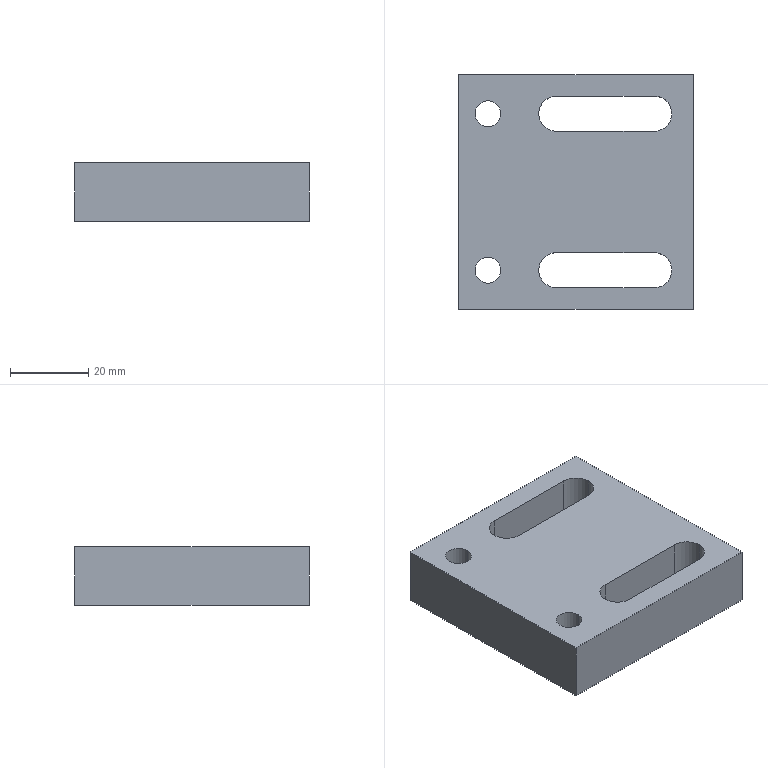Component | SolidWorks | CylinderSupportFrame01-1 | 1 solid | 26 faces | box 60 x 60 x 15 mm | volume 43488 mm3 | cylinder 14 | plane 12 | commonest cylinder face diameters 9 x6 11 x4 6.6 x4
build123d program:
from build123d import *

# Parameters (mm, degrees)
BOSS_EXTRUDE1_DEPTH                               = 60
SKETCH2_W                                         = 105
SKETCH2_H                                         = 15
BOSS_EXTRUDE2_DEPTH                               = 30
SKETCH5_W                                         = 111.678
SKETCH5_H                                         = 197
CUT_EXTRUDE1_DEPTH                                = 275.853
HOLE_SIZE_ACCORDING_TO_TYPE_OF_HEX_SO_D           = 6.6
HOLE_SIZE_ACCORDING_TO_TYPE_OF_HEX_SO_CBORE_D     = 11
HOLE_SIZE_ACCORDING_TO_TYPE_OF_HEX_SO_CBORE_DEPTH = 6.8
CUT_EXTRUDE2_DEPTH                                = 122.861


with BuildPart() as part:
    # Sketch1 → Boss-Extrude1 (new body)
    with BuildSketch(Plane(origin=(0, 0, 0), x_dir=(1, 0, 0), z_dir=(0, 1, 0))):
        Polygon((45, 0), (105, 0), (105, -15), (60, -15), (60, -197), (150, -197), (150, -212), (45, -212), align=None)
    extrude(amount=BOSS_EXTRUDE1_DEPTH)

    # Sketch2 → Boss-Extrude2 (add)
    with BuildSketch(Plane.XZ):
        with Locations((97.5, 204.5)):
            Rectangle(SKETCH2_W, SKETCH2_H)
    extrude(amount=BOSS_EXTRUDE2_DEPTH)

    # Sketch5 → Cut-Extrude1 (cut, through all)
    with BuildSketch(Plane(origin=(0, 60, 0), x_dir=(1, 0, 0), z_dir=(0, 1, 0))):
        with Locations((94.161, -113.5)):
            Rectangle(SKETCH5_W, SKETCH5_H)
    extrude(amount=-CUT_EXTRUDE1_DEPTH, mode=Mode.SUBTRACT)

    # Hole Size _ according to_ type of Hex So (through all)
    with Locations(Plane(origin=(52.5, 50, 0), x_dir=(-1, 0, 0), z_dir=(0, 0, -1))):
        with Locations((0, 0), (0, -40)):
            CounterBoreHole(HOLE_SIZE_ACCORDING_TO_TYPE_OF_HEX_SO_D / 2, HOLE_SIZE_ACCORDING_TO_TYPE_OF_HEX_SO_CBORE_D / 2, HOLE_SIZE_ACCORDING_TO_TYPE_OF_HEX_SO_CBORE_DEPTH)

    # Sketch7 → Cut-Extrude2 (cut, through all)
    with BuildSketch(Plane.XY.offset(15)):
        with BuildLine():
            Line((95, 5.5), (70, 5.5))
            ThreePointArc((70, 5.5), (65.5, 10), (70, 14.5))
            Line((70, 14.5), (95, 14.5))
            ThreePointArc((95, 14.5), (99.5, 10), (95, 5.5))
        make_face()
    cut_extrude2 = extrude(amount=-CUT_EXTRUDE2_DEPTH, mode=Mode.SUBTRACT)

    # Mirror1: Cut-Extrude2 across plane
    add(cut_extrude2.mirror(Plane.ZX.offset(30)), mode=Mode.SUBTRACT)


solid = part.part

# Placed as in the assembly
solid = solid.moved(Location((-44.66, -15.234, 43.104), (0, 0, 0)))
STEP:
#1=CARTESIAN_POINT('',(1.982,1.546,1.697));
#2=VERTEX_POINT('',#1);
#3=CARTESIAN_POINT('',(2.159,1.369,1.697));
#4=VERTEX_POINT('',#3);
#5=CARTESIAN_POINT('',(1.982,1.369,1.697));
#6=DIRECTION('',(0.,0.,-1.));
#7=DIRECTION('',(1.,0.,0.));
#8=AXIS2_PLACEMENT_3D('',#5,#6,#7);
#9=CIRCLE('',#8,0.1772);
#10=EDGE_CURVE('',#2,#4,#9,.T.);
#11=ORIENTED_EDGE('',*,*,#10,.T.);
#12=CARTESIAN_POINT('',(2.159,1.369,2.288));
#13=VERTEX_POINT('',#12);
#14=CARTESIAN_POINT('',(2.159,1.369,1.697));
#15=DIRECTION('',(0.,0.,1.));
#16=VECTOR('',#15,39.37);
#17=LINE('',#14,#16);
#18=EDGE_CURVE('',#4,#13,#17,.T.);
#19=ORIENTED_EDGE('',*,*,#18,.T.);
#20=CARTESIAN_POINT('',(1.982,1.546,2.288));
#21=VERTEX_POINT('',#20);
#22=CARTESIAN_POINT('',(1.982,1.369,2.288));
#23=DIRECTION('',(0.,0.,-1.));
#24=DIRECTION('',(1.,0.,0.));
#25=AXIS2_PLACEMENT_3D('',#22,#23,#24);
#26=CIRCLE('',#25,0.1772);
#27=EDGE_CURVE('',#21,#13,#26,.T.);
#28=ORIENTED_EDGE('',*,*,#27,.F.);
#29=CARTESIAN_POINT('',(1.982,1.546,1.697));
#30=DIRECTION('',(0.,0.,1.));
#31=VECTOR('',#30,39.37);
#32=LINE('',#29,#31);
#33=EDGE_CURVE('',#2,#21,#32,.T.);
#34=ORIENTED_EDGE('',*,*,#33,.F.);
#35=EDGE_LOOP('',(#11,#19,#28,#34));
#36=FACE_OUTER_BOUND('',#35,.T.);
#37=CARTESIAN_POINT('',(1.982,1.369,1.697));
#38=DIRECTION('',(0.,0.,1.));
#39=DIRECTION('',(1.,0.,0.));
#40=AXIS2_PLACEMENT_3D('',#37,#38,#39);
#41=CYLINDRICAL_SURFACE('',#40,0.1772);
#42=ADVANCED_FACE('',(#36),#41,.F.);
#43=CARTESIAN_POINT('',(2.159,-0.2061,1.697));
#44=VERTEX_POINT('',#43);
#45=CARTESIAN_POINT('',(1.982,-0.0289,1.697));
#46=VERTEX_POINT('',#45);
#47=CARTESIAN_POINT('',(1.982,-0.2061,1.697));
#48=DIRECTION('',(0.,0.,1.));
#49=DIRECTION('',(1.,0.,0.));
#50=AXIS2_PLACEMENT_3D('',#47,#48,#49);
#51=CIRCLE('',#50,0.1772);
#52=EDGE_CURVE('',#44,#46,#51,.T.);
#53=ORIENTED_EDGE('',*,*,#52,.F.);
#54=CARTESIAN_POINT('',(2.159,-0.2061,2.288));
#55=VERTEX_POINT('',#54);
#56=CARTESIAN_POINT('',(2.159,-0.2061,1.697));
#57=DIRECTION('',(0.,0.,1.));
#58=VECTOR('',#57,39.37);
#59=LINE('',#56,#58);
#60=EDGE_CURVE('',#44,#55,#59,.T.);
#61=ORIENTED_EDGE('',*,*,#60,.T.);
#62=CARTESIAN_POINT('',(1.982,-0.0289,2.288));
#63=VERTEX_POINT('',#62);
#64=CARTESIAN_POINT('',(1.982,-0.2061,2.288));
#65=DIRECTION('',(0.,0.,1.));
#66=DIRECTION('',(1.,0.,0.));
#67=AXIS2_PLACEMENT_3D('',#64,#65,#66);
#68=CIRCLE('',#67,0.1772);
#69=EDGE_CURVE('',#55,#63,#68,.T.);
#70=ORIENTED_EDGE('',*,*,#69,.T.);
#71=CARTESIAN_POINT('',(1.982,-0.0289,1.697));
#72=DIRECTION('',(0.,0.,1.));
#73=VECTOR('',#72,39.37);
#74=LINE('',#71,#73);
#75=EDGE_CURVE('',#46,#63,#74,.T.);
#76=ORIENTED_EDGE('',*,*,#75,.F.);
#77=EDGE_LOOP('',(#53,#61,#70,#76));
#78=FACE_OUTER_BOUND('',#77,.T.);
#79=CARTESIAN_POINT('',(1.982,-0.2061,1.697));
#80=DIRECTION('',(0.,0.,1.));
#81=DIRECTION('',(1.,0.,0.));
#82=AXIS2_PLACEMENT_3D('',#79,#80,#81);
#83=CYLINDRICAL_SURFACE('',#82,0.1772);
#84=ADVANCED_FACE('',(#78),#83,.F.);
#85=CARTESIAN_POINT('',(0.5252,1.369,1.965));
#86=VERTEX_POINT('',#85);
#87=CARTESIAN_POINT('',(0.09214,1.369,1.965));
#88=VERTEX_POINT('',#87);
#89=CARTESIAN_POINT('',(0.3087,1.369,1.965));
#90=DIRECTION('',(0.,0.,-1.));
#91=DIRECTION('',(-1.,0.,0.));
#92=AXIS2_PLACEMENT_3D('',#89,#90,#91);
#93=CIRCLE('',#92,0.2165);
#94=EDGE_CURVE('',#86,#88,#93,.T.);
#95=ORIENTED_EDGE('',*,*,#94,.F.);
#96=CARTESIAN_POINT('',(0.5252,1.369,1.697));
#97=VERTEX_POINT('',#96);
#98=CARTESIAN_POINT('',(0.5252,1.369,1.697));
#99=DIRECTION('',(0.,0.,-1.));
#100=VECTOR('',#99,39.37);
#101=LINE('',#98,#100);
#102=EDGE_CURVE('',#86,#97,#101,.T.);
#103=ORIENTED_EDGE('',*,*,#102,.T.);
#104=CARTESIAN_POINT('',(0.09214,1.369,1.697));
#105=VERTEX_POINT('',#104);
#106=CARTESIAN_POINT('',(0.3087,1.369,1.697));
#107=DIRECTION('',(0.,0.,-1.));
#108=DIRECTION('',(-1.,0.,0.));
#109=AXIS2_PLACEMENT_3D('',#106,#107,#108);
#110=CIRCLE('',#109,0.2165);
#111=EDGE_CURVE('',#97,#105,#110,.T.);
#112=ORIENTED_EDGE('',*,*,#111,.T.);
#113=CARTESIAN_POINT('',(0.09214,1.369,1.697));
#114=DIRECTION('',(0.,0.,-1.));
#115=VECTOR('',#114,39.37);
#116=LINE('',#113,#115);
#117=EDGE_CURVE('',#88,#105,#116,.T.);
#118=ORIENTED_EDGE('',*,*,#117,.F.);
#119=EDGE_LOOP('',(#95,#103,#112,#118));
#120=FACE_OUTER_BOUND('',#119,.T.);
#121=CARTESIAN_POINT('',(0.3087,1.369,1.697));
#122=DIRECTION('',(0.,0.,-1.));
#123=DIRECTION('',(-1.,0.,0.));
#124=AXIS2_PLACEMENT_3D('',#121,#122,#123);
#125=CYLINDRICAL_SURFACE('',#124,0.2165);
#126=ADVANCED_FACE('',(#120),#125,.F.);
#127=CARTESIAN_POINT('',(0.4386,1.369,2.288));
#128=VERTEX_POINT('',#127);
#129=CARTESIAN_POINT('',(0.1788,1.369,2.288));
#130=VERTEX_POINT('',#129);
#131=CARTESIAN_POINT('',(0.3087,1.369,2.288));
#132=DIRECTION('',(0.,0.,-1.));
#133=DIRECTION('',(-1.,0.,0.));
#134=AXIS2_PLACEMENT_3D('',#131,#132,#133);
#135=CIRCLE('',#134,0.1299);
#136=EDGE_CURVE('',#128,#130,#135,.T.);
#137=ORIENTED_EDGE('',*,*,#136,.F.);
#138=CARTESIAN_POINT('',(0.4386,1.369,1.965));
#139=VERTEX_POINT('',#138);
#140=CARTESIAN_POINT('',(0.4386,1.369,1.697));
#141=DIRECTION('',(0.,0.,-1.));
#142=VECTOR('',#141,39.37);
#143=LINE('',#140,#142);
#144=EDGE_CURVE('',#128,#139,#143,.T.);
#145=ORIENTED_EDGE('',*,*,#144,.T.);
#146=CARTESIAN_POINT('',(0.1788,1.369,1.965));
#147=VERTEX_POINT('',#146);
#148=CARTESIAN_POINT('',(0.3087,1.369,1.965));
#149=DIRECTION('',(0.,0.,-1.));
#150=DIRECTION('',(-1.,0.,0.));
#151=AXIS2_PLACEMENT_3D('',#148,#149,#150);
#152=CIRCLE('',#151,0.1299);
#153=EDGE_CURVE('',#139,#147,#152,.T.);
#154=ORIENTED_EDGE('',*,*,#153,.T.);
#155=CARTESIAN_POINT('',(0.1788,1.369,1.697));
#156=DIRECTION('',(0.,0.,-1.));
#157=VECTOR('',#156,39.37);
#158=LINE('',#155,#157);
#159=EDGE_CURVE('',#130,#147,#158,.T.);
#160=ORIENTED_EDGE('',*,*,#159,.F.);
#161=EDGE_LOOP('',(#137,#145,#154,#160));
#162=FACE_OUTER_BOUND('',#161,.T.);
#163=CARTESIAN_POINT('',(0.3087,1.369,1.697));
#164=DIRECTION('',(0.,0.,-1.));
#165=DIRECTION('',(-1.,0.,0.));
#166=AXIS2_PLACEMENT_3D('',#163,#164,#165);
#167=CYLINDRICAL_SURFACE('',#166,0.1299);
#168=ADVANCED_FACE('',(#162),#167,.F.);
#169=CARTESIAN_POINT('',(0.5252,-0.2061,1.965));
#170=VERTEX_POINT('',#169);
#171=CARTESIAN_POINT('',(0.09214,-0.2061,1.965));
#172=VERTEX_POINT('',#171);
#173=CARTESIAN_POINT('',(0.3087,-0.2061,1.965));
#174=DIRECTION('',(0.,0.,-1.));
#175=DIRECTION('',(-1.,0.,0.));
#176=AXIS2_PLACEMENT_3D('',#173,#174,#175);
#177=CIRCLE('',#176,0.2165);
#178=EDGE_CURVE('',#170,#172,#177,.T.);
#179=ORIENTED_EDGE('',*,*,#178,.F.);
#180=CARTESIAN_POINT('',(0.5252,-0.2061,1.697));
#181=VERTEX_POINT('',#180);
#182=CARTESIAN_POINT('',(0.5252,-0.2061,1.697));
#183=DIRECTION('',(0.,0.,-1.));
#184=VECTOR('',#183,39.37);
#185=LINE('',#182,#184);
#186=EDGE_CURVE('',#170,#181,#185,.T.);
#187=ORIENTED_EDGE('',*,*,#186,.T.);
#188=CARTESIAN_POINT('',(0.09214,-0.2061,1.697));
#189=VERTEX_POINT('',#188);
#190=CARTESIAN_POINT('',(0.3087,-0.2061,1.697));
#191=DIRECTION('',(0.,0.,-1.));
#192=DIRECTION('',(-1.,0.,0.));
#193=AXIS2_PLACEMENT_3D('',#190,#191,#192);
#194=CIRCLE('',#193,0.2165);
#195=EDGE_CURVE('',#181,#189,#194,.T.);
#196=ORIENTED_EDGE('',*,*,#195,.T.);
#197=CARTESIAN_POINT('',(0.09214,-0.2061,1.697));
#198=DIRECTION('',(0.,0.,-1.));
#199=VECTOR('',#198,39.37);
#200=LINE('',#197,#199);
#201=EDGE_CURVE('',#172,#189,#200,.T.);
#202=ORIENTED_EDGE('',*,*,#201,.F.);
#203=EDGE_LOOP('',(#179,#187,#196,#202));
#204=FACE_OUTER_BOUND('',#203,.T.);
#205=CARTESIAN_POINT('',(0.3087,-0.2061,1.697));
#206=DIRECTION('',(0.,0.,-1.));
#207=DIRECTION('',(-1.,0.,0.));
#208=AXIS2_PLACEMENT_3D('',#205,#206,#207);
#209=CYLINDRICAL_SURFACE('',#208,0.2165);
#210=ADVANCED_FACE('',(#204),#209,.F.);
#211=CARTESIAN_POINT('',(0.4386,-0.2061,2.288));
#212=VERTEX_POINT('',#211);
#213=CARTESIAN_POINT('',(0.1788,-0.2061,2.288));
#214=VERTEX_POINT('',#213);
#215=CARTESIAN_POINT('',(0.3087,-0.2061,2.288));
#216=DIRECTION('',(0.,0.,-1.));
#217=DIRECTION('',(-1.,0.,0.));
#218=AXIS2_PLACEMENT_3D('',#215,#216,#217);
#219=CIRCLE('',#218,0.1299);
#220=EDGE_CURVE('',#212,#214,#219,.T.);
#221=ORIENTED_EDGE('',*,*,#220,.F.);
#222=CARTESIAN_POINT('',(0.4386,-0.2061,1.965));
#223=VERTEX_POINT('',#222);
#224=CARTESIAN_POINT('',(0.4386,-0.2061,1.697));
#225=DIRECTION('',(0.,0.,-1.));
#226=VECTOR('',#225,39.37);
#227=LINE('',#224,#226);
#228=EDGE_CURVE('',#212,#223,#227,.T.);
#229=ORIENTED_EDGE('',*,*,#228,.T.);
#230=CARTESIAN_POINT('',(0.1788,-0.2061,1.965));
#231=VERTEX_POINT('',#230);
#232=CARTESIAN_POINT('',(0.3087,-0.2061,1.965));
#233=DIRECTION('',(0.,0.,-1.));
#234=DIRECTION('',(-1.,0.,0.));
#235=AXIS2_PLACEMENT_3D('',#232,#233,#234);
#236=CIRCLE('',#235,0.1299);
#237=EDGE_CURVE('',#223,#231,#236,.T.);
#238=ORIENTED_EDGE('',*,*,#237,.T.);
#239=CARTESIAN_POINT('',(0.1788,-0.2061,1.697));
#240=DIRECTION('',(0.,0.,-1.));
#241=VECTOR('',#240,39.37);
#242=LINE('',#239,#241);
#243=EDGE_CURVE('',#214,#231,#242,.T.);
#244=ORIENTED_EDGE('',*,*,#243,.F.);
#245=EDGE_LOOP('',(#221,#229,#238,#244));
#246=FACE_OUTER_BOUND('',#245,.T.);
#247=CARTESIAN_POINT('',(0.3087,-0.2061,1.697));
#248=DIRECTION('',(0.,0.,-1.));
#249=DIRECTION('',(-1.,0.,0.));
#250=AXIS2_PLACEMENT_3D('',#247,#248,#249);
#251=CYLINDRICAL_SURFACE('',#250,0.1299);
#252=ADVANCED_FACE('',(#246),#251,.F.);
#253=CARTESIAN_POINT('',(0.0134,-0.5998,2.288));
#254=VERTEX_POINT('',#253);
#255=CARTESIAN_POINT('',(2.376,-0.5998,2.288));
#256=VERTEX_POINT('',#255);
#257=CARTESIAN_POINT('',(0.604,-0.5998,2.288));
#258=DIRECTION('',(1.,0.,0.));
#259=VECTOR('',#258,39.37);
#260=LINE('',#257,#259);
#261=EDGE_CURVE('',#254,#256,#260,.T.);
#262=ORIENTED_EDGE('',*,*,#261,.T.);
#263=CARTESIAN_POINT('',(2.376,1.762,2.288));
#264=VERTEX_POINT('',#263);
#265=CARTESIAN_POINT('',(2.376,1.762,2.288));
#266=DIRECTION('',(0.,-1.,0.));
#267=VECTOR('',#266,39.37);
#268=LINE('',#265,#267);
#269=EDGE_CURVE('',#264,#256,#268,.T.);
#270=ORIENTED_EDGE('',*,*,#269,.F.);
#271=CARTESIAN_POINT('',(0.0134,1.762,2.288));
#272=VERTEX_POINT('',#271);
#273=CARTESIAN_POINT('',(0.604,1.762,2.288));
#274=DIRECTION('',(1.,0.,0.));
#275=VECTOR('',#274,39.37);
#276=LINE('',#273,#275);
#277=EDGE_CURVE('',#272,#264,#276,.T.);
#278=ORIENTED_EDGE('',*,*,#277,.F.);
#279=CARTESIAN_POINT('',(0.0134,1.762,2.288));
#280=DIRECTION('',(0.,1.,0.));
#281=VECTOR('',#280,39.37);
#282=LINE('',#279,#281);
#283=EDGE_CURVE('',#254,#272,#282,.T.);
#284=ORIENTED_EDGE('',*,*,#283,.F.);
#285=EDGE_LOOP('',(#262,#270,#278,#284));
#286=FACE_OUTER_BOUND('',#285,.T.);
#287=CARTESIAN_POINT('',(0.3087,-0.2061,2.288));
#288=DIRECTION('',(0.,0.,-1.));
#289=DIRECTION('',(-1.,0.,0.));
#290=AXIS2_PLACEMENT_3D('',#287,#288,#289);
#291=CIRCLE('',#290,0.1299);
#292=EDGE_CURVE('',#214,#212,#291,.T.);
#293=ORIENTED_EDGE('',*,*,#292,.T.);
#294=ORIENTED_EDGE('',*,*,#220,.T.);
#295=EDGE_LOOP('',(#293,#294));
#296=FACE_BOUND('',#295,.T.);
#297=CARTESIAN_POINT('',(0.3087,1.369,2.288));
#298=DIRECTION('',(0.,0.,-1.));
#299=DIRECTION('',(-1.,0.,0.));
#300=AXIS2_PLACEMENT_3D('',#297,#298,#299);
#301=CIRCLE('',#300,0.1299);
#302=EDGE_CURVE('',#130,#128,#301,.T.);
#303=ORIENTED_EDGE('',*,*,#302,.T.);
#304=ORIENTED_EDGE('',*,*,#136,.T.);
#305=EDGE_LOOP('',(#303,#304));
#306=FACE_BOUND('',#305,.T.);
#307=CARTESIAN_POINT('',(0.9977,-0.0289,2.288));
#308=VERTEX_POINT('',#307);
#309=CARTESIAN_POINT('',(1.982,-0.0289,2.288));
#310=DIRECTION('',(-1.,-0.,0.));
#311=VECTOR('',#310,39.37);
#312=LINE('',#309,#311);
#313=EDGE_CURVE('',#63,#308,#312,.T.);
#314=ORIENTED_EDGE('',*,*,#313,.F.);
#315=ORIENTED_EDGE('',*,*,#69,.F.);
#316=CARTESIAN_POINT('',(1.982,-0.3832,2.288));
#317=VERTEX_POINT('',#316);
#318=CARTESIAN_POINT('',(1.982,-0.2061,2.288));
#319=DIRECTION('',(0.,0.,1.));
#320=DIRECTION('',(1.,0.,0.));
#321=AXIS2_PLACEMENT_3D('',#318,#319,#320);
#322=CIRCLE('',#321,0.1772);
#323=EDGE_CURVE('',#317,#55,#322,.T.);
#324=ORIENTED_EDGE('',*,*,#323,.F.);
#325=CARTESIAN_POINT('',(0.9977,-0.3832,2.288));
#326=VERTEX_POINT('',#325);
#327=CARTESIAN_POINT('',(1.982,-0.3832,2.288));
#328=DIRECTION('',(1.,0.,0.));
#329=VECTOR('',#328,39.37);
#330=LINE('',#327,#329);
#331=EDGE_CURVE('',#326,#317,#330,.T.);
#332=ORIENTED_EDGE('',*,*,#331,.F.);
#333=CARTESIAN_POINT('',(0.9977,-0.2061,2.288));
#334=DIRECTION('',(0.,0.,1.));
#335=DIRECTION('',(1.,0.,0.));
#336=AXIS2_PLACEMENT_3D('',#333,#334,#335);
#337=CIRCLE('',#336,0.1772);
#338=EDGE_CURVE('',#308,#326,#337,.T.);
#339=ORIENTED_EDGE('',*,*,#338,.F.);
#340=EDGE_LOOP('',(#314,#315,#324,#332,#339));
#341=FACE_BOUND('',#340,.T.);
#342=ORIENTED_EDGE('',*,*,#27,.T.);
#343=CARTESIAN_POINT('',(1.982,1.192,2.288));
#344=VERTEX_POINT('',#343);
#345=CARTESIAN_POINT('',(1.982,1.369,2.288));
#346=DIRECTION('',(0.,0.,-1.));
#347=DIRECTION('',(1.,0.,0.));
#348=AXIS2_PLACEMENT_3D('',#345,#346,#347);
#349=CIRCLE('',#348,0.1772);
#350=EDGE_CURVE('',#13,#344,#349,.T.);
#351=ORIENTED_EDGE('',*,*,#350,.T.);
#352=CARTESIAN_POINT('',(0.9977,1.192,2.288));
#353=VERTEX_POINT('',#352);
#354=CARTESIAN_POINT('',(1.982,1.192,2.288));
#355=DIRECTION('',(-1.,0.,0.));
#356=VECTOR('',#355,39.37);
#357=LINE('',#354,#356);
#358=EDGE_CURVE('',#344,#353,#357,.T.);
#359=ORIENTED_EDGE('',*,*,#358,.T.);
#360=CARTESIAN_POINT('',(0.9977,1.546,2.288));
#361=VERTEX_POINT('',#360);
#362=CARTESIAN_POINT('',(0.9977,1.369,2.288));
#363=DIRECTION('',(0.,0.,-1.));
#364=DIRECTION('',(1.,0.,0.));
#365=AXIS2_PLACEMENT_3D('',#362,#363,#364);
#366=CIRCLE('',#365,0.1772);
#367=EDGE_CURVE('',#353,#361,#366,.T.);
#368=ORIENTED_EDGE('',*,*,#367,.T.);
#369=CARTESIAN_POINT('',(1.982,1.546,2.288));
#370=DIRECTION('',(1.,-0.,0.));
#371=VECTOR('',#370,39.37);
#372=LINE('',#369,#371);
#373=EDGE_CURVE('',#361,#21,#372,.T.);
#374=ORIENTED_EDGE('',*,*,#373,.T.);
#375=EDGE_LOOP('',(#342,#351,#359,#368,#374));
#376=FACE_BOUND('',#375,.T.);
#377=CARTESIAN_POINT('',(0.604,1.762,2.288));
#378=DIRECTION('',(0.,0.,-1.));
#379=DIRECTION('',(-1.,0.,0.));
#380=AXIS2_PLACEMENT_3D('',#377,#378,#379);
#381=PLANE('',#380);
#382=ADVANCED_FACE('',(#286,#296,#306,#341,#376),#381,.F.);
#383=CARTESIAN_POINT('',(2.376,-0.5998,1.697));
#384=VERTEX_POINT('',#383);
#385=CARTESIAN_POINT('',(0.0134,-0.5998,1.697));
#386=VERTEX_POINT('',#385);
#387=CARTESIAN_POINT('',(0.0134,-0.5998,1.697));
#388=DIRECTION('',(-1.,0.,0.));
#389=VECTOR('',#388,39.37);
#390=LINE('',#387,#389);
#391=EDGE_CURVE('',#384,#386,#390,.T.);
#392=ORIENTED_EDGE('',*,*,#391,.T.);
#393=CARTESIAN_POINT('',(0.0134,1.762,1.697));
#394=VERTEX_POINT('',#393);
#395=CARTESIAN_POINT('',(0.0134,1.762,1.697));
#396=DIRECTION('',(0.,-1.,0.));
#397=VECTOR('',#396,39.37);
#398=LINE('',#395,#397);
#399=EDGE_CURVE('',#394,#386,#398,.T.);
#400=ORIENTED_EDGE('',*,*,#399,.F.);
#401=CARTESIAN_POINT('',(2.376,1.762,1.697));
#402=VERTEX_POINT('',#401);
#403=CARTESIAN_POINT('',(0.0134,1.762,1.697));
#404=DIRECTION('',(-1.,0.,0.));
#405=VECTOR('',#404,39.37);
#406=LINE('',#403,#405);
#407=EDGE_CURVE('',#402,#394,#406,.T.);
#408=ORIENTED_EDGE('',*,*,#407,.F.);
#409=CARTESIAN_POINT('',(2.376,1.762,1.697));
#410=DIRECTION('',(0.,-1.,0.));
#411=VECTOR('',#410,39.37);
#412=LINE('',#409,#411);
#413=EDGE_CURVE('',#402,#384,#412,.T.);
#414=ORIENTED_EDGE('',*,*,#413,.T.);
#415=EDGE_LOOP('',(#392,#400,#408,#414));
#416=FACE_OUTER_BOUND('',#415,.T.);
#417=CARTESIAN_POINT('',(0.3087,-0.2061,1.697));
#418=DIRECTION('',(0.,0.,-1.));
#419=DIRECTION('',(-1.,0.,0.));
#420=AXIS2_PLACEMENT_3D('',#417,#418,#419);
#421=CIRCLE('',#420,0.2165);
#422=EDGE_CURVE('',#189,#181,#421,.T.);
#423=ORIENTED_EDGE('',*,*,#422,.F.);
#424=ORIENTED_EDGE('',*,*,#195,.F.);
#425=EDGE_LOOP('',(#423,#424));
#426=FACE_BOUND('',#425,.T.);
#427=CARTESIAN_POINT('',(0.3087,1.369,1.697));
#428=DIRECTION('',(0.,0.,-1.));
#429=DIRECTION('',(-1.,0.,0.));
#430=AXIS2_PLACEMENT_3D('',#427,#428,#429);
#431=CIRCLE('',#430,0.2165);
#432=EDGE_CURVE('',#105,#97,#431,.T.);
#433=ORIENTED_EDGE('',*,*,#432,.F.);
#434=ORIENTED_EDGE('',*,*,#111,.F.);
#435=EDGE_LOOP('',(#433,#434));
#436=FACE_BOUND('',#435,.T.);
#437=CARTESIAN_POINT('',(0.9977,-0.3832,1.697));
#438=VERTEX_POINT('',#437);
#439=CARTESIAN_POINT('',(1.982,-0.3832,1.697));
#440=VERTEX_POINT('',#439);
#441=CARTESIAN_POINT('',(1.982,-0.3832,1.697));
#442=DIRECTION('',(1.,0.,0.));
#443=VECTOR('',#442,39.37);
#444=LINE('',#441,#443);
#445=EDGE_CURVE('',#438,#440,#444,.T.);
#446=ORIENTED_EDGE('',*,*,#445,.T.);
#447=CARTESIAN_POINT('',(1.982,-0.2061,1.697));
#448=DIRECTION('',(0.,0.,1.));
#449=DIRECTION('',(1.,0.,0.));
#450=AXIS2_PLACEMENT_3D('',#447,#448,#449);
#451=CIRCLE('',#450,0.1772);
#452=EDGE_CURVE('',#440,#44,#451,.T.);
#453=ORIENTED_EDGE('',*,*,#452,.T.);
#454=ORIENTED_EDGE('',*,*,#52,.T.);
#455=CARTESIAN_POINT('',(0.9977,-0.0289,1.697));
#456=VERTEX_POINT('',#455);
#457=CARTESIAN_POINT('',(1.982,-0.0289,1.697));
#458=DIRECTION('',(-1.,-0.,0.));
#459=VECTOR('',#458,39.37);
#460=LINE('',#457,#459);
#461=EDGE_CURVE('',#46,#456,#460,.T.);
#462=ORIENTED_EDGE('',*,*,#461,.T.);
#463=CARTESIAN_POINT('',(0.9977,-0.2061,1.697));
#464=DIRECTION('',(0.,0.,1.));
#465=DIRECTION('',(1.,0.,0.));
#466=AXIS2_PLACEMENT_3D('',#463,#464,#465);
#467=CIRCLE('',#466,0.1772);
#468=EDGE_CURVE('',#456,#438,#467,.T.);
#469=ORIENTED_EDGE('',*,*,#468,.T.);
#470=EDGE_LOOP('',(#446,#453,#454,#462,#469));
#471=FACE_BOUND('',#470,.T.);
#472=ORIENTED_EDGE('',*,*,#10,.F.);
#473=CARTESIAN_POINT('',(0.9977,1.546,1.697));
#474=VERTEX_POINT('',#473);
#475=CARTESIAN_POINT('',(1.982,1.546,1.697));
#476=DIRECTION('',(1.,-0.,0.));
#477=VECTOR('',#476,39.37);
#478=LINE('',#475,#477);
#479=EDGE_CURVE('',#474,#2,#478,.T.);
#480=ORIENTED_EDGE('',*,*,#479,.F.);
#481=CARTESIAN_POINT('',(0.9977,1.192,1.697));
#482=VERTEX_POINT('',#481);
#483=CARTESIAN_POINT('',(0.9977,1.369,1.697));
#484=DIRECTION('',(0.,0.,-1.));
#485=DIRECTION('',(1.,0.,0.));
#486=AXIS2_PLACEMENT_3D('',#483,#484,#485);
#487=CIRCLE('',#486,0.1772);
#488=EDGE_CURVE('',#482,#474,#487,.T.);
#489=ORIENTED_EDGE('',*,*,#488,.F.);
#490=CARTESIAN_POINT('',(1.982,1.192,1.697));
#491=VERTEX_POINT('',#490);
#492=CARTESIAN_POINT('',(1.982,1.192,1.697));
#493=DIRECTION('',(-1.,0.,0.));
#494=VECTOR('',#493,39.37);
#495=LINE('',#492,#494);
#496=EDGE_CURVE('',#491,#482,#495,.T.);
#497=ORIENTED_EDGE('',*,*,#496,.F.);
#498=CARTESIAN_POINT('',(1.982,1.369,1.697));
#499=DIRECTION('',(0.,0.,-1.));
#500=DIRECTION('',(1.,0.,0.));
#501=AXIS2_PLACEMENT_3D('',#498,#499,#500);
#502=CIRCLE('',#501,0.1772);
#503=EDGE_CURVE('',#4,#491,#502,.T.);
#504=ORIENTED_EDGE('',*,*,#503,.F.);
#505=EDGE_LOOP('',(#472,#480,#489,#497,#504));
#506=FACE_BOUND('',#505,.T.);
#507=CARTESIAN_POINT('',(0.0134,1.762,1.697));
#508=DIRECTION('',(0.,0.,1.));
#509=DIRECTION('',(1.,0.,0.));
#510=AXIS2_PLACEMENT_3D('',#507,#508,#509);
#511=PLANE('',#510);
#512=ADVANCED_FACE('',(#416,#426,#436,#471,#506),#511,.F.);
#513=CARTESIAN_POINT('',(2.376,-0.5998,2.288));
#514=DIRECTION('',(0.,0.,-1.));
#515=VECTOR('',#514,39.37);
#516=LINE('',#513,#515);
#517=EDGE_CURVE('',#256,#384,#516,.T.);
#518=ORIENTED_EDGE('',*,*,#517,.T.);
#519=ORIENTED_EDGE('',*,*,#413,.F.);
#520=CARTESIAN_POINT('',(2.376,1.762,2.288));
#521=DIRECTION('',(0.,0.,-1.));
#522=VECTOR('',#521,39.37);
#523=LINE('',#520,#522);
#524=EDGE_CURVE('',#264,#402,#523,.T.);
#525=ORIENTED_EDGE('',*,*,#524,.F.);
#526=ORIENTED_EDGE('',*,*,#269,.T.);
#527=EDGE_LOOP('',(#518,#519,#525,#526));
#528=FACE_OUTER_BOUND('',#527,.T.);
#529=CARTESIAN_POINT('',(2.376,1.762,2.288));
#530=DIRECTION('',(-1.,0.,0.));
#531=DIRECTION('',(0.,0.,1.));
#532=AXIS2_PLACEMENT_3D('',#529,#530,#531);
#533=PLANE('',#532);
#534=ADVANCED_FACE('',(#528),#533,.F.);
#535=CARTESIAN_POINT('',(0.0134,-0.5998,1.697));
#536=DIRECTION('',(0.,0.,1.));
#537=VECTOR('',#536,39.37);
#538=LINE('',#535,#537);
#539=EDGE_CURVE('',#386,#254,#538,.T.);
#540=ORIENTED_EDGE('',*,*,#539,.T.);
#541=ORIENTED_EDGE('',*,*,#283,.T.);
#542=CARTESIAN_POINT('',(0.0134,1.762,1.697));
#543=DIRECTION('',(0.,0.,1.));
#544=VECTOR('',#543,39.37);
#545=LINE('',#542,#544);
#546=EDGE_CURVE('',#394,#272,#545,.T.);
#547=ORIENTED_EDGE('',*,*,#546,.F.);
#548=ORIENTED_EDGE('',*,*,#399,.T.);
#549=EDGE_LOOP('',(#540,#541,#547,#548));
#550=FACE_OUTER_BOUND('',#549,.T.);
#551=CARTESIAN_POINT('',(0.0134,1.762,1.697));
#552=DIRECTION('',(1.,0.,-0.));
#553=DIRECTION('',(-0.,0.,-1.));
#554=AXIS2_PLACEMENT_3D('',#551,#552,#553);
#555=PLANE('',#554);
#556=ADVANCED_FACE('',(#550),#555,.F.);
#557=ORIENTED_EDGE('',*,*,#546,.T.);
#558=ORIENTED_EDGE('',*,*,#277,.T.);
#559=ORIENTED_EDGE('',*,*,#524,.T.);
#560=ORIENTED_EDGE('',*,*,#407,.T.);
#561=EDGE_LOOP('',(#557,#558,#559,#560));
#562=FACE_OUTER_BOUND('',#561,.T.);
#563=CARTESIAN_POINT('',(-1.758,1.762,1.697));
#564=DIRECTION('',(0.,-1.,0.));
#565=DIRECTION('',(0.,0.,-1.));
#566=AXIS2_PLACEMENT_3D('',#563,#564,#565);
#567=PLANE('',#566);
#568=ADVANCED_FACE('',(#562),#567,.F.);
#569=ORIENTED_EDGE('',*,*,#261,.F.);
#570=ORIENTED_EDGE('',*,*,#539,.F.);
#571=ORIENTED_EDGE('',*,*,#391,.F.);
#572=ORIENTED_EDGE('',*,*,#517,.F.);
#573=EDGE_LOOP('',(#569,#570,#571,#572));
#574=FACE_OUTER_BOUND('',#573,.T.);
#575=CARTESIAN_POINT('',(-1.758,-0.5998,1.697));
#576=DIRECTION('',(0.,-1.,0.));
#577=DIRECTION('',(0.,0.,-1.));
#578=AXIS2_PLACEMENT_3D('',#575,#576,#577);
#579=PLANE('',#578);
#580=ADVANCED_FACE('',(#574),#579,.T.);
#581=ORIENTED_EDGE('',*,*,#228,.F.);
#582=ORIENTED_EDGE('',*,*,#292,.F.);
#583=ORIENTED_EDGE('',*,*,#243,.T.);
#584=CARTESIAN_POINT('',(0.3087,-0.2061,1.965));
#585=DIRECTION('',(0.,0.,-1.));
#586=DIRECTION('',(-1.,0.,0.));
#587=AXIS2_PLACEMENT_3D('',#584,#585,#586);
#588=CIRCLE('',#587,0.1299);
#589=EDGE_CURVE('',#231,#223,#588,.T.);
#590=ORIENTED_EDGE('',*,*,#589,.T.);
#591=EDGE_LOOP('',(#581,#582,#583,#590));
#592=FACE_OUTER_BOUND('',#591,.T.);
#593=CARTESIAN_POINT('',(0.3087,-0.2061,1.697));
#594=DIRECTION('',(0.,0.,-1.));
#595=DIRECTION('',(-1.,0.,0.));
#596=AXIS2_PLACEMENT_3D('',#593,#594,#595);
#597=CYLINDRICAL_SURFACE('',#596,0.1299);
#598=ADVANCED_FACE('',(#592),#597,.F.);
#599=ORIENTED_EDGE('',*,*,#589,.F.);
#600=ORIENTED_EDGE('',*,*,#237,.F.);
#601=EDGE_LOOP('',(#599,#600));
#602=FACE_BOUND('',#601,.T.);
#603=CARTESIAN_POINT('',(0.3087,-0.2061,1.965));
#604=DIRECTION('',(0.,0.,-1.));
#605=DIRECTION('',(-1.,0.,0.));
#606=AXIS2_PLACEMENT_3D('',#603,#604,#605);
#607=CIRCLE('',#606,0.2165);
#608=EDGE_CURVE('',#172,#170,#607,.T.);
#609=ORIENTED_EDGE('',*,*,#608,.T.);
#610=ORIENTED_EDGE('',*,*,#178,.T.);
#611=EDGE_LOOP('',(#609,#610));
#612=FACE_OUTER_BOUND('',#611,.T.);
#613=CARTESIAN_POINT('',(0.4386,-0.2061,1.965));
#614=DIRECTION('',(0.,0.,1.));
#615=DIRECTION('',(1.,0.,0.));
#616=AXIS2_PLACEMENT_3D('',#613,#614,#615);
#617=PLANE('',#616);
#618=ADVANCED_FACE('',(#602,#612),#617,.F.);
#619=ORIENTED_EDGE('',*,*,#186,.F.);
#620=ORIENTED_EDGE('',*,*,#608,.F.);
#621=ORIENTED_EDGE('',*,*,#201,.T.);
#622=ORIENTED_EDGE('',*,*,#422,.T.);
#623=EDGE_LOOP('',(#619,#620,#621,#622));
#624=FACE_OUTER_BOUND('',#623,.T.);
#625=CARTESIAN_POINT('',(0.3087,-0.2061,1.697));
#626=DIRECTION('',(0.,0.,-1.));
#627=DIRECTION('',(-1.,0.,0.));
#628=AXIS2_PLACEMENT_3D('',#625,#626,#627);
#629=CYLINDRICAL_SURFACE('',#628,0.2165);
#630=ADVANCED_FACE('',(#624),#629,.F.);
#631=ORIENTED_EDGE('',*,*,#144,.F.);
#632=ORIENTED_EDGE('',*,*,#302,.F.);
#633=ORIENTED_EDGE('',*,*,#159,.T.);
#634=CARTESIAN_POINT('',(0.3087,1.369,1.965));
#635=DIRECTION('',(0.,0.,-1.));
#636=DIRECTION('',(-1.,0.,0.));
#637=AXIS2_PLACEMENT_3D('',#634,#635,#636);
#638=CIRCLE('',#637,0.1299);
#639=EDGE_CURVE('',#147,#139,#638,.T.);
#640=ORIENTED_EDGE('',*,*,#639,.T.);
#641=EDGE_LOOP('',(#631,#632,#633,#640));
#642=FACE_OUTER_BOUND('',#641,.T.);
#643=CARTESIAN_POINT('',(0.3087,1.369,1.697));
#644=DIRECTION('',(0.,0.,-1.));
#645=DIRECTION('',(-1.,0.,0.));
#646=AXIS2_PLACEMENT_3D('',#643,#644,#645);
#647=CYLINDRICAL_SURFACE('',#646,0.1299);
#648=ADVANCED_FACE('',(#642),#647,.F.);
#649=ORIENTED_EDGE('',*,*,#639,.F.);
#650=ORIENTED_EDGE('',*,*,#153,.F.);
#651=EDGE_LOOP('',(#649,#650));
#652=FACE_BOUND('',#651,.T.);
#653=CARTESIAN_POINT('',(0.3087,1.369,1.965));
#654=DIRECTION('',(0.,0.,-1.));
#655=DIRECTION('',(-1.,0.,0.));
#656=AXIS2_PLACEMENT_3D('',#653,#654,#655);
#657=CIRCLE('',#656,0.2165);
#658=EDGE_CURVE('',#88,#86,#657,.T.);
#659=ORIENTED_EDGE('',*,*,#658,.T.);
#660=ORIENTED_EDGE('',*,*,#94,.T.);
#661=EDGE_LOOP('',(#659,#660));
#662=FACE_OUTER_BOUND('',#661,.T.);
#663=CARTESIAN_POINT('',(0.4386,1.369,1.965));
#664=DIRECTION('',(0.,0.,1.));
#665=DIRECTION('',(1.,0.,0.));
#666=AXIS2_PLACEMENT_3D('',#663,#664,#665);
#667=PLANE('',#666);
#668=ADVANCED_FACE('',(#652,#662),#667,.F.);
#669=ORIENTED_EDGE('',*,*,#102,.F.);
#670=ORIENTED_EDGE('',*,*,#658,.F.);
#671=ORIENTED_EDGE('',*,*,#117,.T.);
#672=ORIENTED_EDGE('',*,*,#432,.T.);
#673=EDGE_LOOP('',(#669,#670,#671,#672));
#674=FACE_OUTER_BOUND('',#673,.T.);
#675=CARTESIAN_POINT('',(0.3087,1.369,1.697));
#676=DIRECTION('',(0.,0.,-1.));
#677=DIRECTION('',(-1.,0.,0.));
#678=AXIS2_PLACEMENT_3D('',#675,#676,#677);
#679=CYLINDRICAL_SURFACE('',#678,0.2165);
#680=ADVANCED_FACE('',(#674),#679,.F.);
#681=ORIENTED_EDGE('',*,*,#60,.F.);
#682=ORIENTED_EDGE('',*,*,#452,.F.);
#683=CARTESIAN_POINT('',(1.982,-0.3832,1.697));
#684=DIRECTION('',(0.,0.,1.));
#685=VECTOR('',#684,39.37);
#686=LINE('',#683,#685);
#687=EDGE_CURVE('',#440,#317,#686,.T.);
#688=ORIENTED_EDGE('',*,*,#687,.T.);
#689=ORIENTED_EDGE('',*,*,#323,.T.);
#690=EDGE_LOOP('',(#681,#682,#688,#689));
#691=FACE_OUTER_BOUND('',#690,.T.);
#692=CARTESIAN_POINT('',(1.982,-0.2061,1.697));
#693=DIRECTION('',(0.,0.,1.));
#694=DIRECTION('',(1.,0.,0.));
#695=AXIS2_PLACEMENT_3D('',#692,#693,#694);
#696=CYLINDRICAL_SURFACE('',#695,0.1772);
#697=ADVANCED_FACE('',(#691),#696,.F.);
#698=ORIENTED_EDGE('',*,*,#331,.T.);
#699=ORIENTED_EDGE('',*,*,#687,.F.);
#700=ORIENTED_EDGE('',*,*,#445,.F.);
#701=CARTESIAN_POINT('',(0.9977,-0.3832,1.697));
#702=DIRECTION('',(0.,0.,1.));
#703=VECTOR('',#702,39.37);
#704=LINE('',#701,#703);
#705=EDGE_CURVE('',#438,#326,#704,.T.);
#706=ORIENTED_EDGE('',*,*,#705,.T.);
#707=EDGE_LOOP('',(#698,#699,#700,#706));
#708=FACE_OUTER_BOUND('',#707,.T.);
#709=CARTESIAN_POINT('',(1.982,-0.3832,1.697));
#710=DIRECTION('',(0.,-1.,0.));
#711=DIRECTION('',(1.,0.,0.));
#712=AXIS2_PLACEMENT_3D('',#709,#710,#711);
#713=PLANE('',#712);
#714=ADVANCED_FACE('',(#708),#713,.F.);
#715=ORIENTED_EDGE('',*,*,#338,.T.);
#716=ORIENTED_EDGE('',*,*,#705,.F.);
#717=ORIENTED_EDGE('',*,*,#468,.F.);
#718=CARTESIAN_POINT('',(0.9977,-0.0289,1.697));
#719=DIRECTION('',(0.,0.,1.));
#720=VECTOR('',#719,39.37);
#721=LINE('',#718,#720);
#722=EDGE_CURVE('',#456,#308,#721,.T.);
#723=ORIENTED_EDGE('',*,*,#722,.T.);
#724=EDGE_LOOP('',(#715,#716,#717,#723));
#725=FACE_OUTER_BOUND('',#724,.T.);
#726=CARTESIAN_POINT('',(0.9977,-0.2061,1.697));
#727=DIRECTION('',(0.,0.,1.));
#728=DIRECTION('',(1.,0.,0.));
#729=AXIS2_PLACEMENT_3D('',#726,#727,#728);
#730=CYLINDRICAL_SURFACE('',#729,0.1772);
#731=ADVANCED_FACE('',(#725),#730,.F.);
#732=ORIENTED_EDGE('',*,*,#313,.T.);
#733=ORIENTED_EDGE('',*,*,#722,.F.);
#734=ORIENTED_EDGE('',*,*,#461,.F.);
#735=ORIENTED_EDGE('',*,*,#75,.T.);
#736=EDGE_LOOP('',(#732,#733,#734,#735));
#737=FACE_OUTER_BOUND('',#736,.T.);
#738=CARTESIAN_POINT('',(1.982,-0.0289,1.697));
#739=DIRECTION('',(-0.,1.,0.));
#740=DIRECTION('',(-1.,-0.,0.));
#741=AXIS2_PLACEMENT_3D('',#738,#739,#740);
#742=PLANE('',#741);
#743=ADVANCED_FACE('',(#737),#742,.F.);
#744=ORIENTED_EDGE('',*,*,#18,.F.);
#745=ORIENTED_EDGE('',*,*,#503,.T.);
#746=CARTESIAN_POINT('',(1.982,1.192,1.697));
#747=DIRECTION('',(0.,0.,1.));
#748=VECTOR('',#747,39.37);
#749=LINE('',#746,#748);
#750=EDGE_CURVE('',#491,#344,#749,.T.);
#751=ORIENTED_EDGE('',*,*,#750,.T.);
#752=ORIENTED_EDGE('',*,*,#350,.F.);
#753=EDGE_LOOP('',(#744,#745,#751,#752));
#754=FACE_OUTER_BOUND('',#753,.T.);
#755=CARTESIAN_POINT('',(1.982,1.369,1.697));
#756=DIRECTION('',(0.,0.,1.));
#757=DIRECTION('',(1.,0.,0.));
#758=AXIS2_PLACEMENT_3D('',#755,#756,#757);
#759=CYLINDRICAL_SURFACE('',#758,0.1772);
#760=ADVANCED_FACE('',(#754),#759,.F.);
#761=ORIENTED_EDGE('',*,*,#358,.F.);
#762=ORIENTED_EDGE('',*,*,#750,.F.);
#763=ORIENTED_EDGE('',*,*,#496,.T.);
#764=CARTESIAN_POINT('',(0.9977,1.192,1.697));
#765=DIRECTION('',(0.,0.,1.));
#766=VECTOR('',#765,39.37);
#767=LINE('',#764,#766);
#768=EDGE_CURVE('',#482,#353,#767,.T.);
#769=ORIENTED_EDGE('',*,*,#768,.T.);
#770=EDGE_LOOP('',(#761,#762,#763,#769));
#771=FACE_OUTER_BOUND('',#770,.T.);
#772=CARTESIAN_POINT('',(1.982,1.192,1.697));
#773=DIRECTION('',(0.,1.,0.));
#774=DIRECTION('',(-1.,0.,0.));
#775=AXIS2_PLACEMENT_3D('',#772,#773,#774);
#776=PLANE('',#775);
#777=ADVANCED_FACE('',(#771),#776,.T.);
#778=ORIENTED_EDGE('',*,*,#367,.F.);
#779=ORIENTED_EDGE('',*,*,#768,.F.);
#780=ORIENTED_EDGE('',*,*,#488,.T.);
#781=CARTESIAN_POINT('',(0.9977,1.546,1.697));
#782=DIRECTION('',(0.,0.,1.));
#783=VECTOR('',#782,39.37);
#784=LINE('',#781,#783);
#785=EDGE_CURVE('',#474,#361,#784,.T.);
#786=ORIENTED_EDGE('',*,*,#785,.T.);
#787=EDGE_LOOP('',(#778,#779,#780,#786));
#788=FACE_OUTER_BOUND('',#787,.T.);
#789=CARTESIAN_POINT('',(0.9977,1.369,1.697));
#790=DIRECTION('',(0.,0.,1.));
#791=DIRECTION('',(1.,0.,0.));
#792=AXIS2_PLACEMENT_3D('',#789,#790,#791);
#793=CYLINDRICAL_SURFACE('',#792,0.1772);
#794=ADVANCED_FACE('',(#788),#793,.F.);
#795=ORIENTED_EDGE('',*,*,#373,.F.);
#796=ORIENTED_EDGE('',*,*,#785,.F.);
#797=ORIENTED_EDGE('',*,*,#479,.T.);
#798=ORIENTED_EDGE('',*,*,#33,.T.);
#799=EDGE_LOOP('',(#795,#796,#797,#798));
#800=FACE_OUTER_BOUND('',#799,.T.);
#801=CARTESIAN_POINT('',(1.982,1.546,1.697));
#802=DIRECTION('',(-0.,-1.,0.));
#803=DIRECTION('',(1.,-0.,0.));
#804=AXIS2_PLACEMENT_3D('',#801,#802,#803);
#805=PLANE('',#804);
#806=ADVANCED_FACE('',(#800),#805,.T.);
#807=CLOSED_SHELL('',(#42,#84,#126,#168,#210,#252,#382,#512,#534,#556,#568,#580,#598,#618,#630,#648,#668,#680,#697,#714,#731,#743,#760,#777,#794,#806));
#808=MANIFOLD_SOLID_BREP('',#807);
#809=CARTESIAN_POINT('',(0.,0.,0.));
#810=DIRECTION('',(0.,0.,1.));
#811=DIRECTION('',(1.,0.,0.));
#812=AXIS2_PLACEMENT_3D('',#809,#810,#811);
#813=(LENGTH_UNIT()NAMED_UNIT(*)SI_UNIT($,.METRE.));
#814=LENGTH_MEASURE_WITH_UNIT(LENGTH_MEASURE(0.0254),#813);
#815=DIMENSIONAL_EXPONENTS(1.,0.,0.,0.,0.,0.,0.);
#816=(CONVERSION_BASED_UNIT('',#814)LENGTH_UNIT()NAMED_UNIT(#815));
#817=UNCERTAINTY_MEASURE_WITH_UNIT(LENGTH_MEASURE(0.00001),#816,'','');
#818=(NAMED_UNIT(*)PLANE_ANGLE_UNIT()SI_UNIT($,.RADIAN.));
#819=(NAMED_UNIT(*)SI_UNIT($,.STERADIAN.)SOLID_ANGLE_UNIT());
#820=(GEOMETRIC_REPRESENTATION_CONTEXT(3)GLOBAL_UNCERTAINTY_ASSIGNED_CONTEXT((#817))GLOBAL_UNIT_ASSIGNED_CONTEXT((#816,#818,#819))REPRESENTATION_CONTEXT('',''));
#821=ADVANCED_BREP_SHAPE_REPRESENTATION('',(#808,#812),#820);
#822=COLOUR_RGB('',0.7922,0.8196,0.9333);
#823=FILL_AREA_STYLE_COLOUR('',#822);
#824=FILL_AREA_STYLE('',(#823));
#825=SURFACE_STYLE_FILL_AREA(#824);
#826=SURFACE_SIDE_STYLE('',(#825));
#827=SURFACE_STYLE_USAGE(.BOTH.,#826);
#828=PRESENTATION_STYLE_ASSIGNMENT((#827));
#829=STYLED_ITEM('',(#828),#808);
#830=PRESENTATION_LAYER_ASSIGNMENT('','',(#829));
#831=(LENGTH_UNIT()NAMED_UNIT(*)SI_UNIT($,.METRE.));
#832=LENGTH_MEASURE_WITH_UNIT(LENGTH_MEASURE(0.0254),#831);
#833=DIMENSIONAL_EXPONENTS(1.,0.,0.,0.,0.,0.,0.);
#834=(CONVERSION_BASED_UNIT('',#832)LENGTH_UNIT()NAMED_UNIT(#833));
#835=UNCERTAINTY_MEASURE_WITH_UNIT(LENGTH_MEASURE(0.00001),#834,'','');
#836=(NAMED_UNIT(*)PLANE_ANGLE_UNIT()SI_UNIT($,.RADIAN.));
#837=(NAMED_UNIT(*)SI_UNIT($,.STERADIAN.)SOLID_ANGLE_UNIT());
#838=(GEOMETRIC_REPRESENTATION_CONTEXT(3)GLOBAL_UNCERTAINTY_ASSIGNED_CONTEXT((#835))GLOBAL_UNIT_ASSIGNED_CONTEXT((#834,#836,#837))REPRESENTATION_CONTEXT('',''));
#839=MECHANICAL_DESIGN_GEOMETRIC_PRESENTATION_REPRESENTATION('',(#829),#838);